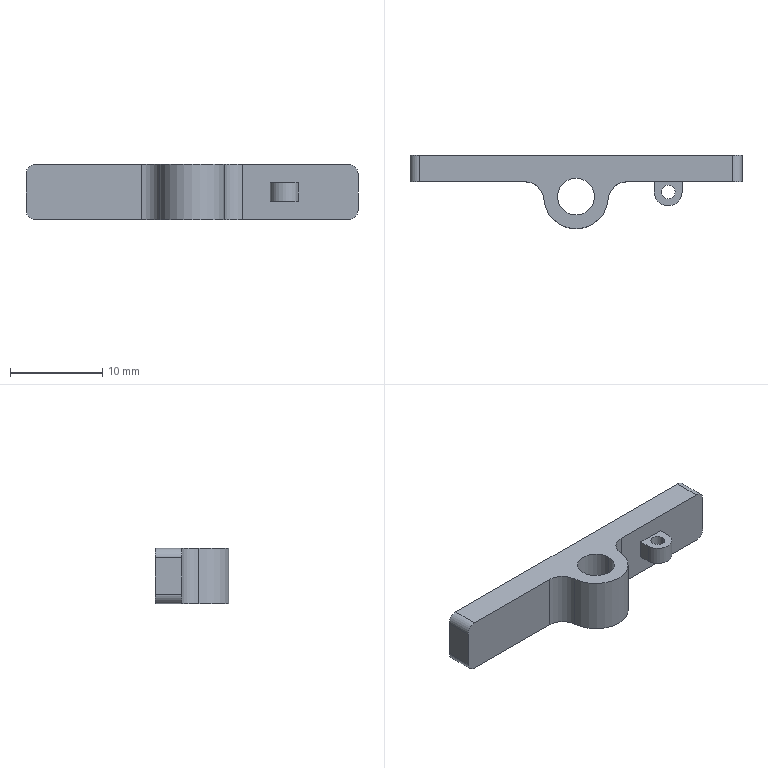Component | SolidWorks | SAWH02-03110A0StopBlock1-1 | 1 solid | 23 faces | box 36 x 8 x 6 mm | volume 751 mm3 | cylinder 12 | plane 11 | commonest cylinder face diameters 4 x4 2 x4 1.5 x2 3 x1 7 x1 | material SUS304
build123d program:
from build123d import *

# Parameters (mm, degrees)
SKETCH1_R           = 2
SKETCH1_R_2         = 0.75
BOSS_EXTRUDE1_DEPTH = 3
FILLET1_R           = 1
SKETCH2_W           = 3
SKETCH2_H           = 2
CUT_EXTRUDE1_DEPTH  = 19.948


with BuildPart() as part:
    # Sketch1 → Boss-Extrude1 (new, symmetric)
    with BuildSketch(Plane.XY):
        with BuildLine():
            Line((-18, 4.5), (18, 4.5))
            Line((18, 4.5), (18, 1.6))
            Line((18, 1.6), (11.5, 1.6))
            Line((11.5, 1.6), (11.5, 0.5))
            ThreePointArc((11.5, 0.5), (10, -1), (8.5, 0.5))
            Line((8.5, 0.5), (8.5, 1.6))
            Line((8.5, 1.6), (5.485, 1.6))
            ThreePointArc((5.485, 1.6), (4.124, 1.065), (3.491, -0.2545))
            ThreePointArc((3.491, -0.2545), (0, -3.5), (-3.491, -0.2545))
            ThreePointArc((-3.491, -0.2545), (-4.124, 1.065), (-5.485, 1.6))
            Line((-5.485, 1.6), (-18, 1.6))
            Line((-18, 1.6), (-18, 4.5))
        make_face()
        Circle(SKETCH1_R, mode=Mode.SUBTRACT)
        with Locations((10, 0.5)):
            Circle(SKETCH1_R_2, mode=Mode.SUBTRACT)
    extrude(amount=BOSS_EXTRUDE1_DEPTH, both=True)

    # Fillet1
    fillet1_edges = [part.edges().sort_by_distance(p)[0] for p in [
        (18, 3.05, 3),
        (-18, 3.05, -3),
        (18, 3.05, -3),
        (-18, 3.05, 3),
    ]]
    fillet(fillet1_edges, radius=FILLET1_R)

    # Sketch2 → Cut-Extrude1 (cut, through all)
    with BuildSketch(Plane.XZ.offset(-1.6)):
        with Locations((10, 2)):
            Rectangle(SKETCH2_W, SKETCH2_H)
        with Locations((10, -2)):
            Rectangle(SKETCH2_W, SKETCH2_H)
    extrude(amount=CUT_EXTRUDE1_DEPTH, mode=Mode.SUBTRACT)


solid = part.part

# Placed as in the assembly
solid = solid.moved(Location((-67.74, 2.612, 37.708), (0, 0, 0)))
STEP:
#1=CARTESIAN_POINT('',(-2.746,0.1028,1.603));
#2=VERTEX_POINT('',#1);
#3=CARTESIAN_POINT('',(-2.588,0.1028,1.603));
#4=VERTEX_POINT('',#3);
#5=CARTESIAN_POINT('',(-2.667,0.1028,1.603));
#6=DIRECTION('',(0.,0.,1.));
#7=DIRECTION('',(1.,0.,0.));
#8=AXIS2_PLACEMENT_3D('',#5,#6,#7);
#9=CIRCLE('',#8,0.07874);
#10=EDGE_CURVE('',#2,#4,#9,.T.);
#11=ORIENTED_EDGE('',*,*,#10,.T.);
#12=CARTESIAN_POINT('',(-2.588,0.1028,1.366));
#13=VERTEX_POINT('',#12);
#14=CARTESIAN_POINT('',(-2.588,0.1028,1.603));
#15=DIRECTION('',(0.,0.,-1.));
#16=VECTOR('',#15,39.37);
#17=LINE('',#14,#16);
#18=EDGE_CURVE('',#4,#13,#17,.T.);
#19=ORIENTED_EDGE('',*,*,#18,.T.);
#20=CARTESIAN_POINT('',(-2.746,0.1028,1.366));
#21=VERTEX_POINT('',#20);
#22=CARTESIAN_POINT('',(-2.667,0.1028,1.366));
#23=DIRECTION('',(0.,0.,1.));
#24=DIRECTION('',(1.,0.,0.));
#25=AXIS2_PLACEMENT_3D('',#22,#23,#24);
#26=CIRCLE('',#25,0.07874);
#27=EDGE_CURVE('',#21,#13,#26,.T.);
#28=ORIENTED_EDGE('',*,*,#27,.F.);
#29=CARTESIAN_POINT('',(-2.746,0.1028,1.603));
#30=DIRECTION('',(0.,0.,-1.));
#31=VECTOR('',#30,39.37);
#32=LINE('',#29,#31);
#33=EDGE_CURVE('',#2,#21,#32,.T.);
#34=ORIENTED_EDGE('',*,*,#33,.F.);
#35=EDGE_LOOP('',(#11,#19,#28,#34));
#36=FACE_OUTER_BOUND('',#35,.T.);
#37=CARTESIAN_POINT('',(-2.667,0.1028,1.603));
#38=DIRECTION('',(0.,0.,-1.));
#39=DIRECTION('',(-1.,0.,0.));
#40=AXIS2_PLACEMENT_3D('',#37,#38,#39);
#41=CYLINDRICAL_SURFACE('',#40,0.07874);
#42=ADVANCED_FACE('',(#36),#41,.F.);
#43=CARTESIAN_POINT('',(-2.303,0.1225,1.524));
#44=VERTEX_POINT('',#43);
#45=CARTESIAN_POINT('',(-2.244,0.1225,1.524));
#46=VERTEX_POINT('',#45);
#47=CARTESIAN_POINT('',(-2.273,0.1225,1.524));
#48=DIRECTION('',(0.,0.,1.));
#49=DIRECTION('',(1.,0.,0.));
#50=AXIS2_PLACEMENT_3D('',#47,#48,#49);
#51=CIRCLE('',#50,0.02953);
#52=EDGE_CURVE('',#44,#46,#51,.T.);
#53=ORIENTED_EDGE('',*,*,#52,.T.);
#54=CARTESIAN_POINT('',(-2.244,0.1225,1.445));
#55=VERTEX_POINT('',#54);
#56=CARTESIAN_POINT('',(-2.244,0.1225,1.603));
#57=DIRECTION('',(0.,0.,-1.));
#58=VECTOR('',#57,39.37);
#59=LINE('',#56,#58);
#60=EDGE_CURVE('',#46,#55,#59,.T.);
#61=ORIENTED_EDGE('',*,*,#60,.T.);
#62=CARTESIAN_POINT('',(-2.303,0.1225,1.445));
#63=VERTEX_POINT('',#62);
#64=CARTESIAN_POINT('',(-2.273,0.1225,1.445));
#65=DIRECTION('',(0.,0.,-1.));
#66=DIRECTION('',(-1.,0.,0.));
#67=AXIS2_PLACEMENT_3D('',#64,#65,#66);
#68=CIRCLE('',#67,0.02953);
#69=EDGE_CURVE('',#55,#63,#68,.T.);
#70=ORIENTED_EDGE('',*,*,#69,.T.);
#71=CARTESIAN_POINT('',(-2.303,0.1225,1.603));
#72=DIRECTION('',(0.,0.,-1.));
#73=VECTOR('',#72,39.37);
#74=LINE('',#71,#73);
#75=EDGE_CURVE('',#44,#63,#74,.T.);
#76=ORIENTED_EDGE('',*,*,#75,.F.);
#77=EDGE_LOOP('',(#53,#61,#70,#76));
#78=FACE_OUTER_BOUND('',#77,.T.);
#79=CARTESIAN_POINT('',(-2.273,0.1225,1.603));
#80=DIRECTION('',(0.,0.,-1.));
#81=DIRECTION('',(-1.,0.,0.));
#82=AXIS2_PLACEMENT_3D('',#79,#80,#81);
#83=CYLINDRICAL_SURFACE('',#82,0.02953);
#84=ADVANCED_FACE('',(#78),#83,.F.);
#85=CARTESIAN_POINT('',(-2.214,0.1225,1.445));
#86=VERTEX_POINT('',#85);
#87=CARTESIAN_POINT('',(-2.332,0.1225,1.445));
#88=VERTEX_POINT('',#87);
#89=CARTESIAN_POINT('',(-2.273,0.1225,1.445));
#90=DIRECTION('',(0.,0.,-1.));
#91=DIRECTION('',(-1.,0.,0.));
#92=AXIS2_PLACEMENT_3D('',#89,#90,#91);
#93=CIRCLE('',#92,0.05906);
#94=EDGE_CURVE('',#86,#88,#93,.T.);
#95=ORIENTED_EDGE('',*,*,#94,.F.);
#96=CARTESIAN_POINT('',(-2.214,0.1225,1.524));
#97=VERTEX_POINT('',#96);
#98=CARTESIAN_POINT('',(-2.214,0.1225,1.603));
#99=DIRECTION('',(0.,0.,-1.));
#100=VECTOR('',#99,39.37);
#101=LINE('',#98,#100);
#102=EDGE_CURVE('',#97,#86,#101,.T.);
#103=ORIENTED_EDGE('',*,*,#102,.F.);
#104=CARTESIAN_POINT('',(-2.332,0.1225,1.524));
#105=VERTEX_POINT('',#104);
#106=CARTESIAN_POINT('',(-2.273,0.1225,1.524));
#107=DIRECTION('',(0.,0.,1.));
#108=DIRECTION('',(1.,0.,0.));
#109=AXIS2_PLACEMENT_3D('',#106,#107,#108);
#110=CIRCLE('',#109,0.05906);
#111=EDGE_CURVE('',#105,#97,#110,.T.);
#112=ORIENTED_EDGE('',*,*,#111,.F.);
#113=CARTESIAN_POINT('',(-2.332,0.1225,1.603));
#114=DIRECTION('',(0.,0.,-1.));
#115=VECTOR('',#114,39.37);
#116=LINE('',#113,#115);
#117=EDGE_CURVE('',#105,#88,#116,.T.);
#118=ORIENTED_EDGE('',*,*,#117,.T.);
#119=EDGE_LOOP('',(#95,#103,#112,#118));
#120=FACE_OUTER_BOUND('',#119,.T.);
#121=CARTESIAN_POINT('',(-2.273,0.1225,1.603));
#122=DIRECTION('',(0.,0.,-1.));
#123=DIRECTION('',(-1.,0.,0.));
#124=AXIS2_PLACEMENT_3D('',#121,#122,#123);
#125=CYLINDRICAL_SURFACE('',#124,0.05906);
#126=ADVANCED_FACE('',(#120),#125,.T.);
#127=CARTESIAN_POINT('',(-2.214,0.1658,1.445));
#128=VERTEX_POINT('',#127);
#129=CARTESIAN_POINT('',(-2.214,-0.03495,1.445));
#130=DIRECTION('',(0.,1.,0.));
#131=VECTOR('',#130,39.37);
#132=LINE('',#129,#131);
#133=EDGE_CURVE('',#86,#128,#132,.T.);
#134=ORIENTED_EDGE('',*,*,#133,.T.);
#135=CARTESIAN_POINT('',(-2.214,0.1658,1.524));
#136=VERTEX_POINT('',#135);
#137=CARTESIAN_POINT('',(-2.214,0.1658,1.603));
#138=DIRECTION('',(0.,0.,-1.));
#139=VECTOR('',#138,39.37);
#140=LINE('',#137,#139);
#141=EDGE_CURVE('',#136,#128,#140,.T.);
#142=ORIENTED_EDGE('',*,*,#141,.F.);
#143=CARTESIAN_POINT('',(-2.214,-0.03495,1.524));
#144=DIRECTION('',(0.,1.,0.));
#145=VECTOR('',#144,39.37);
#146=LINE('',#143,#145);
#147=EDGE_CURVE('',#97,#136,#146,.T.);
#148=ORIENTED_EDGE('',*,*,#147,.F.);
#149=ORIENTED_EDGE('',*,*,#102,.T.);
#150=EDGE_LOOP('',(#134,#142,#148,#149));
#151=FACE_OUTER_BOUND('',#150,.T.);
#152=CARTESIAN_POINT('',(-2.214,0.1225,1.603));
#153=DIRECTION('',(-1.,0.,0.));
#154=DIRECTION('',(0.,0.,1.));
#155=AXIS2_PLACEMENT_3D('',#152,#153,#154);
#156=PLANE('',#155);
#157=ADVANCED_FACE('',(#151),#156,.F.);
#158=CARTESIAN_POINT('',(-2.332,0.1658,1.445));
#159=VERTEX_POINT('',#158);
#160=CARTESIAN_POINT('',(-2.332,-0.03495,1.445));
#161=DIRECTION('',(0.,1.,0.));
#162=VECTOR('',#161,39.37);
#163=LINE('',#160,#162);
#164=EDGE_CURVE('',#88,#159,#163,.T.);
#165=ORIENTED_EDGE('',*,*,#164,.F.);
#166=ORIENTED_EDGE('',*,*,#117,.F.);
#167=CARTESIAN_POINT('',(-2.332,0.1658,1.524));
#168=VERTEX_POINT('',#167);
#169=CARTESIAN_POINT('',(-2.332,-0.03495,1.524));
#170=DIRECTION('',(0.,1.,0.));
#171=VECTOR('',#170,39.37);
#172=LINE('',#169,#171);
#173=EDGE_CURVE('',#105,#168,#172,.T.);
#174=ORIENTED_EDGE('',*,*,#173,.T.);
#175=CARTESIAN_POINT('',(-2.332,0.1658,1.603));
#176=DIRECTION('',(0.,0.,-1.));
#177=VECTOR('',#176,39.37);
#178=LINE('',#175,#177);
#179=EDGE_CURVE('',#168,#159,#178,.T.);
#180=ORIENTED_EDGE('',*,*,#179,.T.);
#181=EDGE_LOOP('',(#165,#166,#174,#180));
#182=FACE_OUTER_BOUND('',#181,.T.);
#183=CARTESIAN_POINT('',(-2.332,0.1225,1.603));
#184=DIRECTION('',(1.,0.,0.));
#185=DIRECTION('',(0.,0.,-1.));
#186=AXIS2_PLACEMENT_3D('',#183,#184,#185);
#187=PLANE('',#186);
#188=ADVANCED_FACE('',(#182),#187,.F.);
#189=ORIENTED_EDGE('',*,*,#60,.F.);
#190=CARTESIAN_POINT('',(-2.273,0.1225,1.524));
#191=DIRECTION('',(0.,0.,1.));
#192=DIRECTION('',(1.,0.,0.));
#193=AXIS2_PLACEMENT_3D('',#190,#191,#192);
#194=CIRCLE('',#193,0.02953);
#195=EDGE_CURVE('',#46,#44,#194,.T.);
#196=ORIENTED_EDGE('',*,*,#195,.T.);
#197=ORIENTED_EDGE('',*,*,#75,.T.);
#198=CARTESIAN_POINT('',(-2.273,0.1225,1.445));
#199=DIRECTION('',(0.,0.,-1.));
#200=DIRECTION('',(-1.,0.,0.));
#201=AXIS2_PLACEMENT_3D('',#198,#199,#200);
#202=CIRCLE('',#201,0.02953);
#203=EDGE_CURVE('',#63,#55,#202,.T.);
#204=ORIENTED_EDGE('',*,*,#203,.T.);
#205=EDGE_LOOP('',(#189,#196,#197,#204));
#206=FACE_OUTER_BOUND('',#205,.T.);
#207=CARTESIAN_POINT('',(-2.273,0.1225,1.603));
#208=DIRECTION('',(0.,0.,-1.));
#209=DIRECTION('',(-1.,0.,0.));
#210=AXIS2_PLACEMENT_3D('',#207,#208,#209);
#211=CYLINDRICAL_SURFACE('',#210,0.02953);
#212=ADVANCED_FACE('',(#206),#211,.F.);
#213=ORIENTED_EDGE('',*,*,#27,.T.);
#214=CARTESIAN_POINT('',(-2.667,0.1028,1.366));
#215=DIRECTION('',(0.,0.,1.));
#216=DIRECTION('',(1.,0.,0.));
#217=AXIS2_PLACEMENT_3D('',#214,#215,#216);
#218=CIRCLE('',#217,0.07874);
#219=EDGE_CURVE('',#13,#21,#218,.T.);
#220=ORIENTED_EDGE('',*,*,#219,.T.);
#221=EDGE_LOOP('',(#213,#220));
#222=FACE_BOUND('',#221,.T.);
#223=CARTESIAN_POINT('',(-1.998,0.28,1.366));
#224=VERTEX_POINT('',#223);
#225=CARTESIAN_POINT('',(-1.998,0.1658,1.366));
#226=VERTEX_POINT('',#225);
#227=CARTESIAN_POINT('',(-1.998,0.1225,1.366));
#228=DIRECTION('',(0.,-1.,0.));
#229=VECTOR('',#228,39.37);
#230=LINE('',#227,#229);
#231=EDGE_CURVE('',#224,#226,#230,.T.);
#232=ORIENTED_EDGE('',*,*,#231,.T.);
#233=CARTESIAN_POINT('',(-2.451,0.1658,1.366));
#234=VERTEX_POINT('',#233);
#235=CARTESIAN_POINT('',(-2.451,0.1658,1.366));
#236=DIRECTION('',(1.,-0.,0.));
#237=VECTOR('',#236,39.37);
#238=LINE('',#235,#237);
#239=EDGE_CURVE('',#234,#226,#238,.T.);
#240=ORIENTED_EDGE('',*,*,#239,.F.);
#241=CARTESIAN_POINT('',(-2.529,0.09283,1.366));
#242=VERTEX_POINT('',#241);
#243=CARTESIAN_POINT('',(-2.451,0.0871,1.366));
#244=DIRECTION('',(0.,0.,-1.));
#245=DIRECTION('',(1.,0.,0.));
#246=AXIS2_PLACEMENT_3D('',#243,#244,#245);
#247=CIRCLE('',#246,0.07874);
#248=EDGE_CURVE('',#242,#234,#247,.T.);
#249=ORIENTED_EDGE('',*,*,#248,.F.);
#250=CARTESIAN_POINT('',(-2.804,0.09283,1.366));
#251=VERTEX_POINT('',#250);
#252=CARTESIAN_POINT('',(-2.667,0.1028,1.366));
#253=DIRECTION('',(0.,0.,1.));
#254=DIRECTION('',(1.,0.,0.));
#255=AXIS2_PLACEMENT_3D('',#252,#253,#254);
#256=CIRCLE('',#255,0.1378);
#257=EDGE_CURVE('',#251,#242,#256,.T.);
#258=ORIENTED_EDGE('',*,*,#257,.F.);
#259=CARTESIAN_POINT('',(-2.883,0.1658,1.366));
#260=VERTEX_POINT('',#259);
#261=CARTESIAN_POINT('',(-2.883,0.0871,1.366));
#262=DIRECTION('',(0.,0.,-1.));
#263=DIRECTION('',(-1.,0.,0.));
#264=AXIS2_PLACEMENT_3D('',#261,#262,#263);
#265=CIRCLE('',#264,0.07874);
#266=EDGE_CURVE('',#260,#251,#265,.T.);
#267=ORIENTED_EDGE('',*,*,#266,.F.);
#268=CARTESIAN_POINT('',(-3.336,0.1658,1.366));
#269=VERTEX_POINT('',#268);
#270=CARTESIAN_POINT('',(-3.376,0.1658,1.366));
#271=DIRECTION('',(1.,-0.,0.));
#272=VECTOR('',#271,39.37);
#273=LINE('',#270,#272);
#274=EDGE_CURVE('',#269,#260,#273,.T.);
#275=ORIENTED_EDGE('',*,*,#274,.F.);
#276=CARTESIAN_POINT('',(-3.336,0.28,1.366));
#277=VERTEX_POINT('',#276);
#278=CARTESIAN_POINT('',(-3.336,0.1225,1.366));
#279=DIRECTION('',(0.,1.,0.));
#280=VECTOR('',#279,39.37);
#281=LINE('',#278,#280);
#282=EDGE_CURVE('',#269,#277,#281,.T.);
#283=ORIENTED_EDGE('',*,*,#282,.T.);
#284=CARTESIAN_POINT('',(-3.376,0.28,1.366));
#285=DIRECTION('',(-1.,0.,0.));
#286=VECTOR('',#285,39.37);
#287=LINE('',#284,#286);
#288=EDGE_CURVE('',#224,#277,#287,.T.);
#289=ORIENTED_EDGE('',*,*,#288,.F.);
#290=EDGE_LOOP('',(#232,#240,#249,#258,#267,#275,#283,#289));
#291=FACE_OUTER_BOUND('',#290,.T.);
#292=CARTESIAN_POINT('',(-2.273,0.1225,1.366));
#293=DIRECTION('',(0.,0.,1.));
#294=DIRECTION('',(1.,0.,0.));
#295=AXIS2_PLACEMENT_3D('',#292,#293,#294);
#296=PLANE('',#295);
#297=ADVANCED_FACE('',(#222,#291),#296,.F.);
#298=ORIENTED_EDGE('',*,*,#10,.F.);
#299=CARTESIAN_POINT('',(-2.667,0.1028,1.603));
#300=DIRECTION('',(0.,0.,1.));
#301=DIRECTION('',(1.,0.,0.));
#302=AXIS2_PLACEMENT_3D('',#299,#300,#301);
#303=CIRCLE('',#302,0.07874);
#304=EDGE_CURVE('',#4,#2,#303,.T.);
#305=ORIENTED_EDGE('',*,*,#304,.F.);
#306=EDGE_LOOP('',(#298,#305));
#307=FACE_BOUND('',#306,.T.);
#308=CARTESIAN_POINT('',(-2.529,0.09283,1.603));
#309=VERTEX_POINT('',#308);
#310=CARTESIAN_POINT('',(-2.451,0.1658,1.603));
#311=VERTEX_POINT('',#310);
#312=CARTESIAN_POINT('',(-2.451,0.0871,1.603));
#313=DIRECTION('',(0.,0.,-1.));
#314=DIRECTION('',(1.,0.,0.));
#315=AXIS2_PLACEMENT_3D('',#312,#313,#314);
#316=CIRCLE('',#315,0.07874);
#317=EDGE_CURVE('',#309,#311,#316,.T.);
#318=ORIENTED_EDGE('',*,*,#317,.T.);
#319=CARTESIAN_POINT('',(-1.998,0.1658,1.603));
#320=VERTEX_POINT('',#319);
#321=CARTESIAN_POINT('',(-2.214,0.1658,1.603));
#322=DIRECTION('',(1.,0.,0.));
#323=VECTOR('',#322,39.37);
#324=LINE('',#321,#323);
#325=EDGE_CURVE('',#311,#320,#324,.T.);
#326=ORIENTED_EDGE('',*,*,#325,.T.);
#327=CARTESIAN_POINT('',(-1.998,0.28,1.603));
#328=VERTEX_POINT('',#327);
#329=CARTESIAN_POINT('',(-1.998,0.28,1.603));
#330=DIRECTION('',(0.,1.,0.));
#331=VECTOR('',#330,39.37);
#332=LINE('',#329,#331);
#333=EDGE_CURVE('',#320,#328,#332,.T.);
#334=ORIENTED_EDGE('',*,*,#333,.T.);
#335=CARTESIAN_POINT('',(-3.336,0.28,1.603));
#336=VERTEX_POINT('',#335);
#337=CARTESIAN_POINT('',(-3.376,0.28,1.603));
#338=DIRECTION('',(-1.,0.,0.));
#339=VECTOR('',#338,39.37);
#340=LINE('',#337,#339);
#341=EDGE_CURVE('',#328,#336,#340,.T.);
#342=ORIENTED_EDGE('',*,*,#341,.T.);
#343=CARTESIAN_POINT('',(-3.336,0.1658,1.603));
#344=VERTEX_POINT('',#343);
#345=CARTESIAN_POINT('',(-3.336,0.1658,1.603));
#346=DIRECTION('',(0.,-1.,0.));
#347=VECTOR('',#346,39.37);
#348=LINE('',#345,#347);
#349=EDGE_CURVE('',#336,#344,#348,.T.);
#350=ORIENTED_EDGE('',*,*,#349,.T.);
#351=CARTESIAN_POINT('',(-2.883,0.1658,1.603));
#352=VERTEX_POINT('',#351);
#353=CARTESIAN_POINT('',(-3.376,0.1658,1.603));
#354=DIRECTION('',(1.,-0.,0.));
#355=VECTOR('',#354,39.37);
#356=LINE('',#353,#355);
#357=EDGE_CURVE('',#344,#352,#356,.T.);
#358=ORIENTED_EDGE('',*,*,#357,.T.);
#359=CARTESIAN_POINT('',(-2.804,0.09283,1.603));
#360=VERTEX_POINT('',#359);
#361=CARTESIAN_POINT('',(-2.883,0.0871,1.603));
#362=DIRECTION('',(0.,0.,-1.));
#363=DIRECTION('',(-1.,0.,0.));
#364=AXIS2_PLACEMENT_3D('',#361,#362,#363);
#365=CIRCLE('',#364,0.07874);
#366=EDGE_CURVE('',#352,#360,#365,.T.);
#367=ORIENTED_EDGE('',*,*,#366,.T.);
#368=CARTESIAN_POINT('',(-2.667,0.1028,1.603));
#369=DIRECTION('',(0.,0.,1.));
#370=DIRECTION('',(1.,0.,0.));
#371=AXIS2_PLACEMENT_3D('',#368,#369,#370);
#372=CIRCLE('',#371,0.1378);
#373=EDGE_CURVE('',#360,#309,#372,.T.);
#374=ORIENTED_EDGE('',*,*,#373,.T.);
#375=EDGE_LOOP('',(#318,#326,#334,#342,#350,#358,#367,#374));
#376=FACE_OUTER_BOUND('',#375,.T.);
#377=CARTESIAN_POINT('',(-2.273,0.1225,1.603));
#378=DIRECTION('',(0.,0.,1.));
#379=DIRECTION('',(1.,0.,0.));
#380=AXIS2_PLACEMENT_3D('',#377,#378,#379);
#381=PLANE('',#380);
#382=ADVANCED_FACE('',(#307,#376),#381,.T.);
#383=CARTESIAN_POINT('',(-1.958,0.1658,1.563));
#384=VERTEX_POINT('',#383);
#385=CARTESIAN_POINT('',(-1.958,0.1658,1.406));
#386=VERTEX_POINT('',#385);
#387=CARTESIAN_POINT('',(-1.958,0.1658,1.603));
#388=DIRECTION('',(0.,0.,-1.));
#389=VECTOR('',#388,39.37);
#390=LINE('',#387,#389);
#391=EDGE_CURVE('',#384,#386,#390,.T.);
#392=ORIENTED_EDGE('',*,*,#391,.T.);
#393=CARTESIAN_POINT('',(-1.958,0.28,1.406));
#394=VERTEX_POINT('',#393);
#395=CARTESIAN_POINT('',(-1.958,0.1658,1.406));
#396=DIRECTION('',(0.,1.,0.));
#397=VECTOR('',#396,39.37);
#398=LINE('',#395,#397);
#399=EDGE_CURVE('',#386,#394,#398,.T.);
#400=ORIENTED_EDGE('',*,*,#399,.T.);
#401=CARTESIAN_POINT('',(-1.958,0.28,1.563));
#402=VERTEX_POINT('',#401);
#403=CARTESIAN_POINT('',(-1.958,0.28,1.603));
#404=DIRECTION('',(0.,0.,-1.));
#405=VECTOR('',#404,39.37);
#406=LINE('',#403,#405);
#407=EDGE_CURVE('',#402,#394,#406,.T.);
#408=ORIENTED_EDGE('',*,*,#407,.F.);
#409=CARTESIAN_POINT('',(-1.958,0.1658,1.563));
#410=DIRECTION('',(0.,-1.,0.));
#411=VECTOR('',#410,39.37);
#412=LINE('',#409,#411);
#413=EDGE_CURVE('',#402,#384,#412,.T.);
#414=ORIENTED_EDGE('',*,*,#413,.T.);
#415=EDGE_LOOP('',(#392,#400,#408,#414));
#416=FACE_OUTER_BOUND('',#415,.T.);
#417=CARTESIAN_POINT('',(-1.958,0.1658,1.603));
#418=DIRECTION('',(-1.,0.,0.));
#419=DIRECTION('',(0.,0.,1.));
#420=AXIS2_PLACEMENT_3D('',#417,#418,#419);
#421=PLANE('',#420);
#422=ADVANCED_FACE('',(#416),#421,.F.);
#423=ORIENTED_EDGE('',*,*,#288,.T.);
#424=CARTESIAN_POINT('',(-3.376,0.28,1.406));
#425=VERTEX_POINT('',#424);
#426=CARTESIAN_POINT('',(-3.336,0.28,1.406));
#427=DIRECTION('',(0.,1.,0.));
#428=DIRECTION('',(0.,0.,-1.));
#429=AXIS2_PLACEMENT_3D('',#426,#427,#428);
#430=CIRCLE('',#429,0.03937);
#431=EDGE_CURVE('',#277,#425,#430,.T.);
#432=ORIENTED_EDGE('',*,*,#431,.T.);
#433=CARTESIAN_POINT('',(-3.376,0.28,1.563));
#434=VERTEX_POINT('',#433);
#435=CARTESIAN_POINT('',(-3.376,0.28,1.603));
#436=DIRECTION('',(0.,0.,-1.));
#437=VECTOR('',#436,39.37);
#438=LINE('',#435,#437);
#439=EDGE_CURVE('',#434,#425,#438,.T.);
#440=ORIENTED_EDGE('',*,*,#439,.F.);
#441=CARTESIAN_POINT('',(-3.336,0.28,1.563));
#442=DIRECTION('',(0.,1.,0.));
#443=DIRECTION('',(0.,0.,-1.));
#444=AXIS2_PLACEMENT_3D('',#441,#442,#443);
#445=CIRCLE('',#444,0.03937);
#446=EDGE_CURVE('',#434,#336,#445,.T.);
#447=ORIENTED_EDGE('',*,*,#446,.T.);
#448=ORIENTED_EDGE('',*,*,#341,.F.);
#449=CARTESIAN_POINT('',(-1.998,0.28,1.563));
#450=DIRECTION('',(0.,1.,0.));
#451=DIRECTION('',(0.,0.,-1.));
#452=AXIS2_PLACEMENT_3D('',#449,#450,#451);
#453=CIRCLE('',#452,0.03937);
#454=EDGE_CURVE('',#328,#402,#453,.T.);
#455=ORIENTED_EDGE('',*,*,#454,.T.);
#456=ORIENTED_EDGE('',*,*,#407,.T.);
#457=CARTESIAN_POINT('',(-1.998,0.28,1.406));
#458=DIRECTION('',(0.,1.,0.));
#459=DIRECTION('',(0.,0.,-1.));
#460=AXIS2_PLACEMENT_3D('',#457,#458,#459);
#461=CIRCLE('',#460,0.03937);
#462=EDGE_CURVE('',#394,#224,#461,.T.);
#463=ORIENTED_EDGE('',*,*,#462,.T.);
#464=EDGE_LOOP('',(#423,#432,#440,#447,#448,#455,#456,#463));
#465=FACE_OUTER_BOUND('',#464,.T.);
#466=CARTESIAN_POINT('',(-3.376,0.28,1.603));
#467=DIRECTION('',(0.,-1.,0.));
#468=DIRECTION('',(0.,0.,-1.));
#469=AXIS2_PLACEMENT_3D('',#466,#467,#468);
#470=PLANE('',#469);
#471=ADVANCED_FACE('',(#465),#470,.F.);
#472=ORIENTED_EDGE('',*,*,#439,.T.);
#473=CARTESIAN_POINT('',(-3.376,0.1658,1.406));
#474=VERTEX_POINT('',#473);
#475=CARTESIAN_POINT('',(-3.376,0.28,1.406));
#476=DIRECTION('',(0.,-1.,0.));
#477=VECTOR('',#476,39.37);
#478=LINE('',#475,#477);
#479=EDGE_CURVE('',#425,#474,#478,.T.);
#480=ORIENTED_EDGE('',*,*,#479,.T.);
#481=CARTESIAN_POINT('',(-3.376,0.1658,1.563));
#482=VERTEX_POINT('',#481);
#483=CARTESIAN_POINT('',(-3.376,0.1658,1.603));
#484=DIRECTION('',(0.,0.,-1.));
#485=VECTOR('',#484,39.37);
#486=LINE('',#483,#485);
#487=EDGE_CURVE('',#482,#474,#486,.T.);
#488=ORIENTED_EDGE('',*,*,#487,.F.);
#489=CARTESIAN_POINT('',(-3.376,0.28,1.563));
#490=DIRECTION('',(0.,1.,0.));
#491=VECTOR('',#490,39.37);
#492=LINE('',#489,#491);
#493=EDGE_CURVE('',#482,#434,#492,.T.);
#494=ORIENTED_EDGE('',*,*,#493,.T.);
#495=EDGE_LOOP('',(#472,#480,#488,#494));
#496=FACE_OUTER_BOUND('',#495,.T.);
#497=CARTESIAN_POINT('',(-3.376,0.28,1.603));
#498=DIRECTION('',(1.,0.,0.));
#499=DIRECTION('',(0.,0.,-1.));
#500=AXIS2_PLACEMENT_3D('',#497,#498,#499);
#501=PLANE('',#500);
#502=ADVANCED_FACE('',(#496),#501,.F.);
#503=ORIENTED_EDGE('',*,*,#487,.T.);
#504=CARTESIAN_POINT('',(-3.336,0.1658,1.406));
#505=DIRECTION('',(-0.,-1.,0.));
#506=DIRECTION('',(-1.,0.,0.));
#507=AXIS2_PLACEMENT_3D('',#504,#505,#506);
#508=CIRCLE('',#507,0.03937);
#509=EDGE_CURVE('',#474,#269,#508,.T.);
#510=ORIENTED_EDGE('',*,*,#509,.T.);
#511=ORIENTED_EDGE('',*,*,#274,.T.);
#512=CARTESIAN_POINT('',(-2.883,0.1658,1.603));
#513=DIRECTION('',(0.,0.,-1.));
#514=VECTOR('',#513,39.37);
#515=LINE('',#512,#514);
#516=EDGE_CURVE('',#352,#260,#515,.T.);
#517=ORIENTED_EDGE('',*,*,#516,.F.);
#518=ORIENTED_EDGE('',*,*,#357,.F.);
#519=CARTESIAN_POINT('',(-3.336,0.1658,1.563));
#520=DIRECTION('',(-0.,-1.,0.));
#521=DIRECTION('',(-1.,0.,0.));
#522=AXIS2_PLACEMENT_3D('',#519,#520,#521);
#523=CIRCLE('',#522,0.03937);
#524=EDGE_CURVE('',#344,#482,#523,.T.);
#525=ORIENTED_EDGE('',*,*,#524,.T.);
#526=EDGE_LOOP('',(#503,#510,#511,#517,#518,#525));
#527=FACE_OUTER_BOUND('',#526,.T.);
#528=CARTESIAN_POINT('',(-3.376,0.1658,1.603));
#529=DIRECTION('',(0.,1.,0.));
#530=DIRECTION('',(-1.,0.,0.));
#531=AXIS2_PLACEMENT_3D('',#528,#529,#530);
#532=PLANE('',#531);
#533=ADVANCED_FACE('',(#527),#532,.F.);
#534=ORIENTED_EDGE('',*,*,#266,.T.);
#535=CARTESIAN_POINT('',(-2.804,0.09283,1.603));
#536=DIRECTION('',(0.,0.,-1.));
#537=VECTOR('',#536,39.37);
#538=LINE('',#535,#537);
#539=EDGE_CURVE('',#360,#251,#538,.T.);
#540=ORIENTED_EDGE('',*,*,#539,.F.);
#541=ORIENTED_EDGE('',*,*,#366,.F.);
#542=ORIENTED_EDGE('',*,*,#516,.T.);
#543=EDGE_LOOP('',(#534,#540,#541,#542));
#544=FACE_OUTER_BOUND('',#543,.T.);
#545=CARTESIAN_POINT('',(-2.883,0.0871,1.603));
#546=DIRECTION('',(0.,0.,-1.));
#547=DIRECTION('',(-1.,0.,0.));
#548=AXIS2_PLACEMENT_3D('',#545,#546,#547);
#549=CYLINDRICAL_SURFACE('',#548,0.07874);
#550=ADVANCED_FACE('',(#544),#549,.F.);
#551=ORIENTED_EDGE('',*,*,#257,.T.);
#552=CARTESIAN_POINT('',(-2.529,0.09283,1.603));
#553=DIRECTION('',(0.,0.,-1.));
#554=VECTOR('',#553,39.37);
#555=LINE('',#552,#554);
#556=EDGE_CURVE('',#309,#242,#555,.T.);
#557=ORIENTED_EDGE('',*,*,#556,.F.);
#558=ORIENTED_EDGE('',*,*,#373,.F.);
#559=ORIENTED_EDGE('',*,*,#539,.T.);
#560=EDGE_LOOP('',(#551,#557,#558,#559));
#561=FACE_OUTER_BOUND('',#560,.T.);
#562=CARTESIAN_POINT('',(-2.667,0.1028,1.603));
#563=DIRECTION('',(0.,0.,-1.));
#564=DIRECTION('',(-1.,0.,0.));
#565=AXIS2_PLACEMENT_3D('',#562,#563,#564);
#566=CYLINDRICAL_SURFACE('',#565,0.1378);
#567=ADVANCED_FACE('',(#561),#566,.T.);
#568=ORIENTED_EDGE('',*,*,#248,.T.);
#569=CARTESIAN_POINT('',(-2.451,0.1658,1.603));
#570=DIRECTION('',(0.,0.,-1.));
#571=VECTOR('',#570,39.37);
#572=LINE('',#569,#571);
#573=EDGE_CURVE('',#311,#234,#572,.T.);
#574=ORIENTED_EDGE('',*,*,#573,.F.);
#575=ORIENTED_EDGE('',*,*,#317,.F.);
#576=ORIENTED_EDGE('',*,*,#556,.T.);
#577=EDGE_LOOP('',(#568,#574,#575,#576));
#578=FACE_OUTER_BOUND('',#577,.T.);
#579=CARTESIAN_POINT('',(-2.451,0.0871,1.603));
#580=DIRECTION('',(0.,0.,-1.));
#581=DIRECTION('',(-1.,0.,0.));
#582=AXIS2_PLACEMENT_3D('',#579,#580,#581);
#583=CYLINDRICAL_SURFACE('',#582,0.07874);
#584=ADVANCED_FACE('',(#578),#583,.F.);
#585=ORIENTED_EDGE('',*,*,#141,.T.);
#586=CARTESIAN_POINT('',(-2.332,0.1658,1.445));
#587=DIRECTION('',(-1.,0.,0.));
#588=VECTOR('',#587,39.37);
#589=LINE('',#586,#588);
#590=EDGE_CURVE('',#128,#159,#589,.T.);
#591=ORIENTED_EDGE('',*,*,#590,.T.);
#592=ORIENTED_EDGE('',*,*,#179,.F.);
#593=CARTESIAN_POINT('',(-2.332,0.1658,1.524));
#594=DIRECTION('',(1.,0.,0.));
#595=VECTOR('',#594,39.37);
#596=LINE('',#593,#595);
#597=EDGE_CURVE('',#168,#136,#596,.T.);
#598=ORIENTED_EDGE('',*,*,#597,.T.);
#599=EDGE_LOOP('',(#585,#591,#592,#598));
#600=FACE_BOUND('',#599,.T.);
#601=ORIENTED_EDGE('',*,*,#239,.T.);
#602=CARTESIAN_POINT('',(-1.998,0.1658,1.406));
#603=DIRECTION('',(0.,-1.,0.));
#604=DIRECTION('',(0.,0.,1.));
#605=AXIS2_PLACEMENT_3D('',#602,#603,#604);
#606=CIRCLE('',#605,0.03937);
#607=EDGE_CURVE('',#226,#386,#606,.T.);
#608=ORIENTED_EDGE('',*,*,#607,.T.);
#609=ORIENTED_EDGE('',*,*,#391,.F.);
#610=CARTESIAN_POINT('',(-1.998,0.1658,1.563));
#611=DIRECTION('',(0.,-1.,0.));
#612=DIRECTION('',(0.,0.,1.));
#613=AXIS2_PLACEMENT_3D('',#610,#611,#612);
#614=CIRCLE('',#613,0.03937);
#615=EDGE_CURVE('',#384,#320,#614,.T.);
#616=ORIENTED_EDGE('',*,*,#615,.T.);
#617=ORIENTED_EDGE('',*,*,#325,.F.);
#618=ORIENTED_EDGE('',*,*,#573,.T.);
#619=EDGE_LOOP('',(#601,#608,#609,#616,#617,#618));
#620=FACE_OUTER_BOUND('',#619,.T.);
#621=CARTESIAN_POINT('',(-2.451,0.1658,1.603));
#622=DIRECTION('',(0.,1.,0.));
#623=DIRECTION('',(-1.,0.,0.));
#624=AXIS2_PLACEMENT_3D('',#621,#622,#623);
#625=PLANE('',#624);
#626=ADVANCED_FACE('',(#600,#620),#625,.F.);
#627=ORIENTED_EDGE('',*,*,#18,.F.);
#628=ORIENTED_EDGE('',*,*,#304,.T.);
#629=ORIENTED_EDGE('',*,*,#33,.T.);
#630=ORIENTED_EDGE('',*,*,#219,.F.);
#631=EDGE_LOOP('',(#627,#628,#629,#630));
#632=FACE_OUTER_BOUND('',#631,.T.);
#633=CARTESIAN_POINT('',(-2.667,0.1028,1.603));
#634=DIRECTION('',(0.,0.,-1.));
#635=DIRECTION('',(-1.,0.,0.));
#636=AXIS2_PLACEMENT_3D('',#633,#634,#635);
#637=CYLINDRICAL_SURFACE('',#636,0.07874);
#638=ADVANCED_FACE('',(#632),#637,.F.);
#639=ORIENTED_EDGE('',*,*,#431,.F.);
#640=ORIENTED_EDGE('',*,*,#282,.F.);
#641=ORIENTED_EDGE('',*,*,#509,.F.);
#642=ORIENTED_EDGE('',*,*,#479,.F.);
#643=EDGE_LOOP('',(#639,#640,#641,#642));
#644=FACE_OUTER_BOUND('',#643,.T.);
#645=CARTESIAN_POINT('',(-3.336,0.28,1.406));
#646=DIRECTION('',(0.,-1.,0.));
#647=DIRECTION('',(0.,0.,-1.));
#648=AXIS2_PLACEMENT_3D('',#645,#646,#647);
#649=CYLINDRICAL_SURFACE('',#648,0.03937);
#650=ADVANCED_FACE('',(#644),#649,.T.);
#651=ORIENTED_EDGE('',*,*,#446,.F.);
#652=ORIENTED_EDGE('',*,*,#493,.F.);
#653=ORIENTED_EDGE('',*,*,#524,.F.);
#654=ORIENTED_EDGE('',*,*,#349,.F.);
#655=EDGE_LOOP('',(#651,#652,#653,#654));
#656=FACE_OUTER_BOUND('',#655,.T.);
#657=CARTESIAN_POINT('',(-3.336,0.1225,1.563));
#658=DIRECTION('',(0.,1.,0.));
#659=DIRECTION('',(0.,0.,1.));
#660=AXIS2_PLACEMENT_3D('',#657,#658,#659);
#661=CYLINDRICAL_SURFACE('',#660,0.03937);
#662=ADVANCED_FACE('',(#656),#661,.T.);
#663=ORIENTED_EDGE('',*,*,#607,.F.);
#664=ORIENTED_EDGE('',*,*,#231,.F.);
#665=ORIENTED_EDGE('',*,*,#462,.F.);
#666=ORIENTED_EDGE('',*,*,#399,.F.);
#667=EDGE_LOOP('',(#663,#664,#665,#666));
#668=FACE_OUTER_BOUND('',#667,.T.);
#669=CARTESIAN_POINT('',(-1.998,0.1658,1.406));
#670=DIRECTION('',(0.,1.,0.));
#671=DIRECTION('',(0.,0.,1.));
#672=AXIS2_PLACEMENT_3D('',#669,#670,#671);
#673=CYLINDRICAL_SURFACE('',#672,0.03937);
#674=ADVANCED_FACE('',(#668),#673,.T.);
#675=ORIENTED_EDGE('',*,*,#615,.F.);
#676=ORIENTED_EDGE('',*,*,#413,.F.);
#677=ORIENTED_EDGE('',*,*,#454,.F.);
#678=ORIENTED_EDGE('',*,*,#333,.F.);
#679=EDGE_LOOP('',(#675,#676,#677,#678));
#680=FACE_OUTER_BOUND('',#679,.T.);
#681=CARTESIAN_POINT('',(-1.998,0.1225,1.563));
#682=DIRECTION('',(0.,-1.,0.));
#683=DIRECTION('',(0.,0.,-1.));
#684=AXIS2_PLACEMENT_3D('',#681,#682,#683);
#685=CYLINDRICAL_SURFACE('',#684,0.03937);
#686=ADVANCED_FACE('',(#680),#685,.T.);
#687=ORIENTED_EDGE('',*,*,#52,.F.);
#688=ORIENTED_EDGE('',*,*,#195,.F.);
#689=EDGE_LOOP('',(#687,#688));
#690=FACE_BOUND('',#689,.T.);
#691=ORIENTED_EDGE('',*,*,#111,.T.);
#692=ORIENTED_EDGE('',*,*,#147,.T.);
#693=ORIENTED_EDGE('',*,*,#597,.F.);
#694=ORIENTED_EDGE('',*,*,#173,.F.);
#695=EDGE_LOOP('',(#691,#692,#693,#694));
#696=FACE_OUTER_BOUND('',#695,.T.);
#697=CARTESIAN_POINT('',(-2.332,-0.03495,1.524));
#698=DIRECTION('',(0.,0.,1.));
#699=DIRECTION('',(1.,0.,0.));
#700=AXIS2_PLACEMENT_3D('',#697,#698,#699);
#701=PLANE('',#700);
#702=ADVANCED_FACE('',(#690,#696),#701,.T.);
#703=ORIENTED_EDGE('',*,*,#203,.F.);
#704=ORIENTED_EDGE('',*,*,#69,.F.);
#705=EDGE_LOOP('',(#703,#704));
#706=FACE_BOUND('',#705,.T.);
#707=ORIENTED_EDGE('',*,*,#94,.T.);
#708=ORIENTED_EDGE('',*,*,#164,.T.);
#709=ORIENTED_EDGE('',*,*,#590,.F.);
#710=ORIENTED_EDGE('',*,*,#133,.F.);
#711=EDGE_LOOP('',(#707,#708,#709,#710));
#712=FACE_OUTER_BOUND('',#711,.T.);
#713=CARTESIAN_POINT('',(-2.332,-0.03495,1.445));
#714=DIRECTION('',(0.,0.,-1.));
#715=DIRECTION('',(-1.,0.,0.));
#716=AXIS2_PLACEMENT_3D('',#713,#714,#715);
#717=PLANE('',#716);
#718=ADVANCED_FACE('',(#706,#712),#717,.T.);
#719=CLOSED_SHELL('',(#42,#84,#126,#157,#188,#212,#297,#382,#422,#471,#502,#533,#550,#567,#584,#626,#638,#650,#662,#674,#686,#702,#718));
#720=MANIFOLD_SOLID_BREP('',#719);
#721=CARTESIAN_POINT('',(0.,0.,0.));
#722=DIRECTION('',(0.,0.,1.));
#723=DIRECTION('',(1.,0.,0.));
#724=AXIS2_PLACEMENT_3D('',#721,#722,#723);
#725=(LENGTH_UNIT()NAMED_UNIT(*)SI_UNIT($,.METRE.));
#726=LENGTH_MEASURE_WITH_UNIT(LENGTH_MEASURE(0.0254),#725);
#727=DIMENSIONAL_EXPONENTS(1.,0.,0.,0.,0.,0.,0.);
#728=(CONVERSION_BASED_UNIT('',#726)LENGTH_UNIT()NAMED_UNIT(#727));
#729=UNCERTAINTY_MEASURE_WITH_UNIT(LENGTH_MEASURE(0.00001),#728,'','');
#730=(NAMED_UNIT(*)PLANE_ANGLE_UNIT()SI_UNIT($,.RADIAN.));
#731=(NAMED_UNIT(*)SI_UNIT($,.STERADIAN.)SOLID_ANGLE_UNIT());
#732=(GEOMETRIC_REPRESENTATION_CONTEXT(3)GLOBAL_UNCERTAINTY_ASSIGNED_CONTEXT((#729))GLOBAL_UNIT_ASSIGNED_CONTEXT((#728,#730,#731))REPRESENTATION_CONTEXT('',''));
#733=ADVANCED_BREP_SHAPE_REPRESENTATION('',(#720,#724),#732);
#734=COLOUR_RGB('',0.7922,0.8196,0.9333);
#735=FILL_AREA_STYLE_COLOUR('',#734);
#736=FILL_AREA_STYLE('',(#735));
#737=SURFACE_STYLE_FILL_AREA(#736);
#738=SURFACE_SIDE_STYLE('',(#737));
#739=SURFACE_STYLE_USAGE(.BOTH.,#738);
#740=PRESENTATION_STYLE_ASSIGNMENT((#739));
#741=STYLED_ITEM('',(#740),#720);
#742=PRESENTATION_LAYER_ASSIGNMENT('','',(#741));
#743=(LENGTH_UNIT()NAMED_UNIT(*)SI_UNIT($,.METRE.));
#744=LENGTH_MEASURE_WITH_UNIT(LENGTH_MEASURE(0.0254),#743);
#745=DIMENSIONAL_EXPONENTS(1.,0.,0.,0.,0.,0.,0.);
#746=(CONVERSION_BASED_UNIT('',#744)LENGTH_UNIT()NAMED_UNIT(#745));
#747=UNCERTAINTY_MEASURE_WITH_UNIT(LENGTH_MEASURE(0.00001),#746,'','');
#748=(NAMED_UNIT(*)PLANE_ANGLE_UNIT()SI_UNIT($,.RADIAN.));
#749=(NAMED_UNIT(*)SI_UNIT($,.STERADIAN.)SOLID_ANGLE_UNIT());
#750=(GEOMETRIC_REPRESENTATION_CONTEXT(3)GLOBAL_UNCERTAINTY_ASSIGNED_CONTEXT((#747))GLOBAL_UNIT_ASSIGNED_CONTEXT((#746,#748,#749))REPRESENTATION_CONTEXT('',''));
#751=MECHANICAL_DESIGN_GEOMETRIC_PRESENTATION_REPRESENTATION('',(#741),#750);